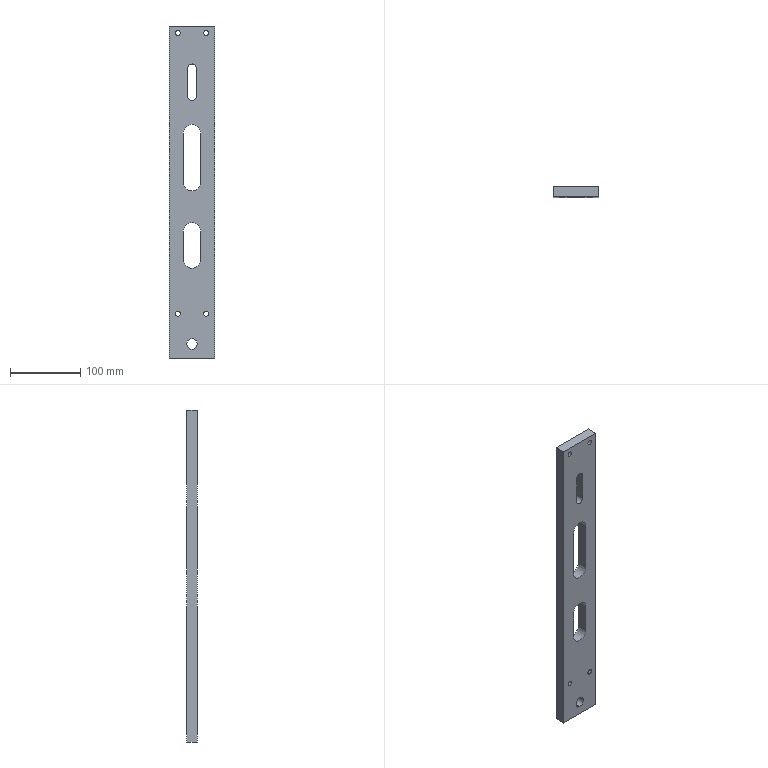Component | SolidWorks | TractionUpperPlate-2 | 1 solid | 31 faces | box 65 x 15 x 473 mm | volume 391343 mm3 | cylinder 19 | plane 12 | commonest cylinder face diameters 7 x8 25 x6 12 x3 15 x2
build123d program:
from build123d import *

# Parameters (mm, degrees)
SKETCH1_W      = 473
SKETCH1_H      = 65
SKETCH1_R      = 3.5
SKETCH1_R_2    = 7.5
EXTRUDE1_DEPTH = 15


with BuildPart() as part:
    # Sketch1 → Extrude1 (new body)
    with BuildSketch(Plane.XY):
        Rectangle(SKETCH1_W, SKETCH1_H)
        with Locations((-226.5, 20)):
            Circle(SKETCH1_R, mode=Mode.SUBTRACT)
        with Locations((-226.5, -20)):
            Circle(SKETCH1_R, mode=Mode.SUBTRACT)
        with Locations((173.5, 20)):
            Circle(SKETCH1_R, mode=Mode.SUBTRACT)
        with Locations((173.5, -20)):
            Circle(SKETCH1_R, mode=Mode.SUBTRACT)
        with Locations((216.5, 0)):
            Circle(SKETCH1_R_2, mode=Mode.SUBTRACT)
        with BuildLine():
            Line((-176.5, 6), (-136.5, 6))
            ThreePointArc((-136.5, 6), (-130.5, 0), (-136.5, -6))
            Line((-136.5, -6), (-176.5, -6))
            ThreePointArc((-176.5, -6), (-182.5, 0), (-176.5, 6))
        make_face(mode=Mode.SUBTRACT)
        with BuildLine():
            Line((-84, 12.5), (-14, 12.5))
            ThreePointArc((-14, 12.5), (-1.5, 0), (-14, -12.5))
            Line((-14, -12.5), (-84, -12.5))
            ThreePointArc((-84, -12.5), (-96.5, 0), (-84, 12.5))
        make_face(mode=Mode.SUBTRACT)
        with BuildLine():
            Line((56, 12.5), (96, 12.5))
            ThreePointArc((96, 12.5), (108.5, 0), (96, -12.5))
            Line((96, -12.5), (56, -12.5))
            ThreePointArc((56, -12.5), (43.5, 0), (56, 12.5))
        make_face(mode=Mode.SUBTRACT)
    extrude(amount=EXTRUDE1_DEPTH)


solid = part.part

# Placed as in the assembly
solid = solid.moved(Location((250.216, 526.983, 40), (90, 0, -90)))
STEP:
#1=CARTESIAN_POINT('',(9.851,20.157,-6.654));
#2=VERTEX_POINT('',#1);
#3=CARTESIAN_POINT('',(9.851,20.157,-7.244));
#4=VERTEX_POINT('',#3);
#5=CARTESIAN_POINT('',(9.851,20.157,-6.949));
#6=DIRECTION('',(0.,-1.,0.));
#7=DIRECTION('',(0.,0.,-1.));
#8=AXIS2_PLACEMENT_3D('',#5,#6,#7);
#9=CIRCLE('',#8,0.2953);
#10=EDGE_CURVE('',#2,#4,#9,.T.);
#11=ORIENTED_EDGE('',*,*,#10,.T.);
#12=CARTESIAN_POINT('',(9.851,20.747,-7.244));
#13=VERTEX_POINT('',#12);
#14=CARTESIAN_POINT('',(9.851,20.157,-7.244));
#15=DIRECTION('',(0.,1.,0.));
#16=VECTOR('',#15,39.37);
#17=LINE('',#14,#16);
#18=EDGE_CURVE('',#4,#13,#17,.T.);
#19=ORIENTED_EDGE('',*,*,#18,.T.);
#20=CARTESIAN_POINT('',(9.851,20.747,-6.654));
#21=VERTEX_POINT('',#20);
#22=CARTESIAN_POINT('',(9.851,20.747,-6.949));
#23=DIRECTION('',(0.,-1.,0.));
#24=DIRECTION('',(0.,0.,-1.));
#25=AXIS2_PLACEMENT_3D('',#22,#23,#24);
#26=CIRCLE('',#25,0.2953);
#27=EDGE_CURVE('',#21,#13,#26,.T.);
#28=ORIENTED_EDGE('',*,*,#27,.F.);
#29=CARTESIAN_POINT('',(9.851,20.157,-6.654));
#30=DIRECTION('',(0.,1.,0.));
#31=VECTOR('',#30,39.37);
#32=LINE('',#29,#31);
#33=EDGE_CURVE('',#2,#21,#32,.T.);
#34=ORIENTED_EDGE('',*,*,#33,.F.);
#35=EDGE_LOOP('',(#11,#19,#28,#34));
#36=FACE_OUTER_BOUND('',#35,.T.);
#37=CARTESIAN_POINT('',(9.851,20.157,-6.949));
#38=DIRECTION('',(0.,1.,0.));
#39=DIRECTION('',(0.,0.,1.));
#40=AXIS2_PLACEMENT_3D('',#37,#38,#39);
#41=CYLINDRICAL_SURFACE('',#40,0.2953);
#42=ADVANCED_FACE('',(#36),#41,.F.);
#43=CARTESIAN_POINT('',(9.064,20.157,-5.118));
#44=VERTEX_POINT('',#43);
#45=CARTESIAN_POINT('',(9.064,20.157,-5.394));
#46=VERTEX_POINT('',#45);
#47=CARTESIAN_POINT('',(9.064,20.157,-5.256));
#48=DIRECTION('',(0.,-1.,0.));
#49=DIRECTION('',(0.,0.,-1.));
#50=AXIS2_PLACEMENT_3D('',#47,#48,#49);
#51=CIRCLE('',#50,0.1378);
#52=EDGE_CURVE('',#44,#46,#51,.T.);
#53=ORIENTED_EDGE('',*,*,#52,.T.);
#54=CARTESIAN_POINT('',(9.064,20.747,-5.394));
#55=VERTEX_POINT('',#54);
#56=CARTESIAN_POINT('',(9.064,20.157,-5.394));
#57=DIRECTION('',(0.,1.,0.));
#58=VECTOR('',#57,39.37);
#59=LINE('',#56,#58);
#60=EDGE_CURVE('',#46,#55,#59,.T.);
#61=ORIENTED_EDGE('',*,*,#60,.T.);
#62=CARTESIAN_POINT('',(9.064,20.747,-5.118));
#63=VERTEX_POINT('',#62);
#64=CARTESIAN_POINT('',(9.064,20.747,-5.256));
#65=DIRECTION('',(0.,-1.,0.));
#66=DIRECTION('',(0.,0.,-1.));
#67=AXIS2_PLACEMENT_3D('',#64,#65,#66);
#68=CIRCLE('',#67,0.1378);
#69=EDGE_CURVE('',#63,#55,#68,.T.);
#70=ORIENTED_EDGE('',*,*,#69,.F.);
#71=CARTESIAN_POINT('',(9.064,20.157,-5.118));
#72=DIRECTION('',(0.,1.,0.));
#73=VECTOR('',#72,39.37);
#74=LINE('',#71,#73);
#75=EDGE_CURVE('',#44,#63,#74,.T.);
#76=ORIENTED_EDGE('',*,*,#75,.F.);
#77=EDGE_LOOP('',(#53,#61,#70,#76));
#78=FACE_OUTER_BOUND('',#77,.T.);
#79=CARTESIAN_POINT('',(9.064,20.157,-5.256));
#80=DIRECTION('',(0.,1.,0.));
#81=DIRECTION('',(0.,0.,1.));
#82=AXIS2_PLACEMENT_3D('',#79,#80,#81);
#83=CYLINDRICAL_SURFACE('',#82,0.1378);
#84=ADVANCED_FACE('',(#78),#83,.F.);
#85=CARTESIAN_POINT('',(10.638,20.157,-5.118));
#86=VERTEX_POINT('',#85);
#87=CARTESIAN_POINT('',(10.638,20.157,-5.394));
#88=VERTEX_POINT('',#87);
#89=CARTESIAN_POINT('',(10.638,20.157,-5.256));
#90=DIRECTION('',(0.,-1.,0.));
#91=DIRECTION('',(0.,0.,-1.));
#92=AXIS2_PLACEMENT_3D('',#89,#90,#91);
#93=CIRCLE('',#92,0.1378);
#94=EDGE_CURVE('',#86,#88,#93,.T.);
#95=ORIENTED_EDGE('',*,*,#94,.T.);
#96=CARTESIAN_POINT('',(10.638,20.747,-5.394));
#97=VERTEX_POINT('',#96);
#98=CARTESIAN_POINT('',(10.638,20.157,-5.394));
#99=DIRECTION('',(0.,1.,0.));
#100=VECTOR('',#99,39.37);
#101=LINE('',#98,#100);
#102=EDGE_CURVE('',#88,#97,#101,.T.);
#103=ORIENTED_EDGE('',*,*,#102,.T.);
#104=CARTESIAN_POINT('',(10.638,20.747,-5.118));
#105=VERTEX_POINT('',#104);
#106=CARTESIAN_POINT('',(10.638,20.747,-5.256));
#107=DIRECTION('',(0.,-1.,0.));
#108=DIRECTION('',(0.,0.,-1.));
#109=AXIS2_PLACEMENT_3D('',#106,#107,#108);
#110=CIRCLE('',#109,0.1378);
#111=EDGE_CURVE('',#105,#97,#110,.T.);
#112=ORIENTED_EDGE('',*,*,#111,.F.);
#113=CARTESIAN_POINT('',(10.638,20.157,-5.118));
#114=DIRECTION('',(0.,1.,0.));
#115=VECTOR('',#114,39.37);
#116=LINE('',#113,#115);
#117=EDGE_CURVE('',#86,#105,#116,.T.);
#118=ORIENTED_EDGE('',*,*,#117,.F.);
#119=EDGE_LOOP('',(#95,#103,#112,#118));
#120=FACE_OUTER_BOUND('',#119,.T.);
#121=CARTESIAN_POINT('',(10.638,20.157,-5.256));
#122=DIRECTION('',(0.,1.,0.));
#123=DIRECTION('',(0.,0.,1.));
#124=AXIS2_PLACEMENT_3D('',#121,#122,#123);
#125=CYLINDRICAL_SURFACE('',#124,0.1378);
#126=ADVANCED_FACE('',(#120),#125,.F.);
#127=CARTESIAN_POINT('',(10.343,20.157,-0.6299));
#128=VERTEX_POINT('',#127);
#129=CARTESIAN_POINT('',(9.851,20.157,-0.1378));
#130=VERTEX_POINT('',#129);
#131=CARTESIAN_POINT('',(9.851,20.157,-0.6299));
#132=DIRECTION('',(0.,-1.,0.));
#133=DIRECTION('',(0.,0.,-1.));
#134=AXIS2_PLACEMENT_3D('',#131,#132,#133);
#135=CIRCLE('',#134,0.4921);
#136=EDGE_CURVE('',#128,#130,#135,.T.);
#137=ORIENTED_EDGE('',*,*,#136,.T.);
#138=CARTESIAN_POINT('',(9.851,20.747,-0.1378));
#139=VERTEX_POINT('',#138);
#140=CARTESIAN_POINT('',(9.851,20.157,-0.1378));
#141=DIRECTION('',(0.,1.,0.));
#142=VECTOR('',#141,39.37);
#143=LINE('',#140,#142);
#144=EDGE_CURVE('',#130,#139,#143,.T.);
#145=ORIENTED_EDGE('',*,*,#144,.T.);
#146=CARTESIAN_POINT('',(10.343,20.747,-0.6299));
#147=VERTEX_POINT('',#146);
#148=CARTESIAN_POINT('',(9.851,20.747,-0.6299));
#149=DIRECTION('',(0.,-1.,0.));
#150=DIRECTION('',(0.,0.,-1.));
#151=AXIS2_PLACEMENT_3D('',#148,#149,#150);
#152=CIRCLE('',#151,0.4921);
#153=EDGE_CURVE('',#147,#139,#152,.T.);
#154=ORIENTED_EDGE('',*,*,#153,.F.);
#155=CARTESIAN_POINT('',(10.343,20.157,-0.6299));
#156=DIRECTION('',(0.,1.,0.));
#157=VECTOR('',#156,39.37);
#158=LINE('',#155,#157);
#159=EDGE_CURVE('',#128,#147,#158,.T.);
#160=ORIENTED_EDGE('',*,*,#159,.F.);
#161=EDGE_LOOP('',(#137,#145,#154,#160));
#162=FACE_OUTER_BOUND('',#161,.T.);
#163=CARTESIAN_POINT('',(9.851,20.157,-0.6299));
#164=DIRECTION('',(0.,1.,0.));
#165=DIRECTION('',(0.,0.,1.));
#166=AXIS2_PLACEMENT_3D('',#163,#164,#165);
#167=CYLINDRICAL_SURFACE('',#166,0.4921);
#168=ADVANCED_FACE('',(#162),#167,.F.);
#169=CARTESIAN_POINT('',(10.343,20.157,4.882));
#170=VERTEX_POINT('',#169);
#171=CARTESIAN_POINT('',(9.851,20.157,5.374));
#172=VERTEX_POINT('',#171);
#173=CARTESIAN_POINT('',(9.851,20.157,4.882));
#174=DIRECTION('',(0.,-1.,0.));
#175=DIRECTION('',(0.,0.,-1.));
#176=AXIS2_PLACEMENT_3D('',#173,#174,#175);
#177=CIRCLE('',#176,0.4921);
#178=EDGE_CURVE('',#170,#172,#177,.T.);
#179=ORIENTED_EDGE('',*,*,#178,.T.);
#180=CARTESIAN_POINT('',(9.851,20.747,5.374));
#181=VERTEX_POINT('',#180);
#182=CARTESIAN_POINT('',(9.851,20.157,5.374));
#183=DIRECTION('',(0.,1.,0.));
#184=VECTOR('',#183,39.37);
#185=LINE('',#182,#184);
#186=EDGE_CURVE('',#172,#181,#185,.T.);
#187=ORIENTED_EDGE('',*,*,#186,.T.);
#188=CARTESIAN_POINT('',(10.343,20.747,4.882));
#189=VERTEX_POINT('',#188);
#190=CARTESIAN_POINT('',(9.851,20.747,4.882));
#191=DIRECTION('',(0.,-1.,0.));
#192=DIRECTION('',(0.,0.,-1.));
#193=AXIS2_PLACEMENT_3D('',#190,#191,#192);
#194=CIRCLE('',#193,0.4921);
#195=EDGE_CURVE('',#189,#181,#194,.T.);
#196=ORIENTED_EDGE('',*,*,#195,.F.);
#197=CARTESIAN_POINT('',(10.343,20.157,4.882));
#198=DIRECTION('',(0.,1.,0.));
#199=VECTOR('',#198,39.37);
#200=LINE('',#197,#199);
#201=EDGE_CURVE('',#170,#189,#200,.T.);
#202=ORIENTED_EDGE('',*,*,#201,.F.);
#203=EDGE_LOOP('',(#179,#187,#196,#202));
#204=FACE_OUTER_BOUND('',#203,.T.);
#205=CARTESIAN_POINT('',(9.851,20.157,4.882));
#206=DIRECTION('',(0.,1.,0.));
#207=DIRECTION('',(0.,0.,1.));
#208=AXIS2_PLACEMENT_3D('',#205,#206,#207);
#209=CYLINDRICAL_SURFACE('',#208,0.4921);
#210=ADVANCED_FACE('',(#204),#209,.F.);
#211=CARTESIAN_POINT('',(9.064,20.157,10.63));
#212=VERTEX_POINT('',#211);
#213=CARTESIAN_POINT('',(9.064,20.157,10.354));
#214=VERTEX_POINT('',#213);
#215=CARTESIAN_POINT('',(9.064,20.157,10.492));
#216=DIRECTION('',(0.,-1.,0.));
#217=DIRECTION('',(0.,0.,-1.));
#218=AXIS2_PLACEMENT_3D('',#215,#216,#217);
#219=CIRCLE('',#218,0.1378);
#220=EDGE_CURVE('',#212,#214,#219,.T.);
#221=ORIENTED_EDGE('',*,*,#220,.T.);
#222=CARTESIAN_POINT('',(9.064,20.747,10.354));
#223=VERTEX_POINT('',#222);
#224=CARTESIAN_POINT('',(9.064,20.157,10.354));
#225=DIRECTION('',(0.,1.,0.));
#226=VECTOR('',#225,39.37);
#227=LINE('',#224,#226);
#228=EDGE_CURVE('',#214,#223,#227,.T.);
#229=ORIENTED_EDGE('',*,*,#228,.T.);
#230=CARTESIAN_POINT('',(9.064,20.747,10.63));
#231=VERTEX_POINT('',#230);
#232=CARTESIAN_POINT('',(9.064,20.747,10.492));
#233=DIRECTION('',(0.,-1.,0.));
#234=DIRECTION('',(0.,0.,-1.));
#235=AXIS2_PLACEMENT_3D('',#232,#233,#234);
#236=CIRCLE('',#235,0.1378);
#237=EDGE_CURVE('',#231,#223,#236,.T.);
#238=ORIENTED_EDGE('',*,*,#237,.F.);
#239=CARTESIAN_POINT('',(9.064,20.157,10.63));
#240=DIRECTION('',(0.,1.,0.));
#241=VECTOR('',#240,39.37);
#242=LINE('',#239,#241);
#243=EDGE_CURVE('',#212,#231,#242,.T.);
#244=ORIENTED_EDGE('',*,*,#243,.F.);
#245=EDGE_LOOP('',(#221,#229,#238,#244));
#246=FACE_OUTER_BOUND('',#245,.T.);
#247=CARTESIAN_POINT('',(9.064,20.157,10.492));
#248=DIRECTION('',(0.,1.,0.));
#249=DIRECTION('',(0.,0.,1.));
#250=AXIS2_PLACEMENT_3D('',#247,#248,#249);
#251=CYLINDRICAL_SURFACE('',#250,0.1378);
#252=ADVANCED_FACE('',(#246),#251,.F.);
#253=CARTESIAN_POINT('',(10.638,20.157,10.63));
#254=VERTEX_POINT('',#253);
#255=CARTESIAN_POINT('',(10.638,20.157,10.354));
#256=VERTEX_POINT('',#255);
#257=CARTESIAN_POINT('',(10.638,20.157,10.492));
#258=DIRECTION('',(0.,-1.,0.));
#259=DIRECTION('',(0.,0.,-1.));
#260=AXIS2_PLACEMENT_3D('',#257,#258,#259);
#261=CIRCLE('',#260,0.1378);
#262=EDGE_CURVE('',#254,#256,#261,.T.);
#263=ORIENTED_EDGE('',*,*,#262,.T.);
#264=CARTESIAN_POINT('',(10.638,20.747,10.354));
#265=VERTEX_POINT('',#264);
#266=CARTESIAN_POINT('',(10.638,20.157,10.354));
#267=DIRECTION('',(0.,1.,0.));
#268=VECTOR('',#267,39.37);
#269=LINE('',#266,#268);
#270=EDGE_CURVE('',#256,#265,#269,.T.);
#271=ORIENTED_EDGE('',*,*,#270,.T.);
#272=CARTESIAN_POINT('',(10.638,20.747,10.63));
#273=VERTEX_POINT('',#272);
#274=CARTESIAN_POINT('',(10.638,20.747,10.492));
#275=DIRECTION('',(0.,-1.,0.));
#276=DIRECTION('',(0.,0.,-1.));
#277=AXIS2_PLACEMENT_3D('',#274,#275,#276);
#278=CIRCLE('',#277,0.1378);
#279=EDGE_CURVE('',#273,#265,#278,.T.);
#280=ORIENTED_EDGE('',*,*,#279,.F.);
#281=CARTESIAN_POINT('',(10.638,20.157,10.63));
#282=DIRECTION('',(0.,1.,0.));
#283=VECTOR('',#282,39.37);
#284=LINE('',#281,#283);
#285=EDGE_CURVE('',#254,#273,#284,.T.);
#286=ORIENTED_EDGE('',*,*,#285,.F.);
#287=EDGE_LOOP('',(#263,#271,#280,#286));
#288=FACE_OUTER_BOUND('',#287,.T.);
#289=CARTESIAN_POINT('',(10.638,20.157,10.492));
#290=DIRECTION('',(0.,1.,0.));
#291=DIRECTION('',(0.,0.,1.));
#292=AXIS2_PLACEMENT_3D('',#289,#290,#291);
#293=CYLINDRICAL_SURFACE('',#292,0.1378);
#294=ADVANCED_FACE('',(#288),#293,.F.);
#295=CARTESIAN_POINT('',(10.087,20.157,8.524));
#296=VERTEX_POINT('',#295);
#297=CARTESIAN_POINT('',(9.851,20.157,8.76));
#298=VERTEX_POINT('',#297);
#299=CARTESIAN_POINT('',(9.851,20.157,8.524));
#300=DIRECTION('',(0.,-1.,0.));
#301=DIRECTION('',(0.,0.,-1.));
#302=AXIS2_PLACEMENT_3D('',#299,#300,#301);
#303=CIRCLE('',#302,0.2362);
#304=EDGE_CURVE('',#296,#298,#303,.T.);
#305=ORIENTED_EDGE('',*,*,#304,.T.);
#306=CARTESIAN_POINT('',(9.851,20.747,8.76));
#307=VERTEX_POINT('',#306);
#308=CARTESIAN_POINT('',(9.851,20.157,8.76));
#309=DIRECTION('',(0.,1.,0.));
#310=VECTOR('',#309,39.37);
#311=LINE('',#308,#310);
#312=EDGE_CURVE('',#298,#307,#311,.T.);
#313=ORIENTED_EDGE('',*,*,#312,.T.);
#314=CARTESIAN_POINT('',(10.087,20.747,8.524));
#315=VERTEX_POINT('',#314);
#316=CARTESIAN_POINT('',(9.851,20.747,8.524));
#317=DIRECTION('',(0.,-1.,0.));
#318=DIRECTION('',(0.,0.,-1.));
#319=AXIS2_PLACEMENT_3D('',#316,#317,#318);
#320=CIRCLE('',#319,0.2362);
#321=EDGE_CURVE('',#315,#307,#320,.T.);
#322=ORIENTED_EDGE('',*,*,#321,.F.);
#323=CARTESIAN_POINT('',(10.087,20.157,8.524));
#324=DIRECTION('',(0.,1.,0.));
#325=VECTOR('',#324,39.37);
#326=LINE('',#323,#325);
#327=EDGE_CURVE('',#296,#315,#326,.T.);
#328=ORIENTED_EDGE('',*,*,#327,.F.);
#329=EDGE_LOOP('',(#305,#313,#322,#328));
#330=FACE_OUTER_BOUND('',#329,.T.);
#331=CARTESIAN_POINT('',(9.851,20.157,8.524));
#332=DIRECTION('',(0.,1.,0.));
#333=DIRECTION('',(0.,0.,1.));
#334=AXIS2_PLACEMENT_3D('',#331,#332,#333);
#335=CYLINDRICAL_SURFACE('',#334,0.2362);
#336=ADVANCED_FACE('',(#330),#335,.F.);
#337=ORIENTED_EDGE('',*,*,#52,.F.);
#338=CARTESIAN_POINT('',(9.064,20.157,-5.256));
#339=DIRECTION('',(0.,-1.,0.));
#340=DIRECTION('',(0.,0.,-1.));
#341=AXIS2_PLACEMENT_3D('',#338,#339,#340);
#342=CIRCLE('',#341,0.1378);
#343=EDGE_CURVE('',#46,#44,#342,.T.);
#344=ORIENTED_EDGE('',*,*,#343,.F.);
#345=EDGE_LOOP('',(#337,#344));
#346=FACE_BOUND('',#345,.T.);
#347=CARTESIAN_POINT('',(9.359,20.157,-0.6299));
#348=VERTEX_POINT('',#347);
#349=CARTESIAN_POINT('',(9.359,20.157,-2.205));
#350=VERTEX_POINT('',#349);
#351=CARTESIAN_POINT('',(9.359,20.157,-0.6299));
#352=DIRECTION('',(0.,0.,-1.));
#353=VECTOR('',#352,39.37);
#354=LINE('',#351,#353);
#355=EDGE_CURVE('',#348,#350,#354,.T.);
#356=ORIENTED_EDGE('',*,*,#355,.F.);
#357=CARTESIAN_POINT('',(9.851,20.157,-0.6299));
#358=DIRECTION('',(0.,-1.,0.));
#359=DIRECTION('',(0.,0.,-1.));
#360=AXIS2_PLACEMENT_3D('',#357,#358,#359);
#361=CIRCLE('',#360,0.4921);
#362=EDGE_CURVE('',#130,#348,#361,.T.);
#363=ORIENTED_EDGE('',*,*,#362,.F.);
#364=ORIENTED_EDGE('',*,*,#136,.F.);
#365=CARTESIAN_POINT('',(10.343,20.157,-2.205));
#366=VERTEX_POINT('',#365);
#367=CARTESIAN_POINT('',(10.343,20.157,-0.6299));
#368=DIRECTION('',(-0.,0.,1.));
#369=VECTOR('',#368,39.37);
#370=LINE('',#367,#369);
#371=EDGE_CURVE('',#366,#128,#370,.T.);
#372=ORIENTED_EDGE('',*,*,#371,.F.);
#373=CARTESIAN_POINT('',(9.851,20.157,-2.205));
#374=DIRECTION('',(0.,-1.,0.));
#375=DIRECTION('',(0.,0.,-1.));
#376=AXIS2_PLACEMENT_3D('',#373,#374,#375);
#377=CIRCLE('',#376,0.4921);
#378=EDGE_CURVE('',#350,#366,#377,.T.);
#379=ORIENTED_EDGE('',*,*,#378,.F.);
#380=EDGE_LOOP('',(#356,#363,#364,#372,#379));
#381=FACE_BOUND('',#380,.T.);
#382=CARTESIAN_POINT('',(9.359,20.157,4.882));
#383=VERTEX_POINT('',#382);
#384=CARTESIAN_POINT('',(9.359,20.157,2.126));
#385=VERTEX_POINT('',#384);
#386=CARTESIAN_POINT('',(9.359,20.157,4.882));
#387=DIRECTION('',(0.,0.,-1.));
#388=VECTOR('',#387,39.37);
#389=LINE('',#386,#388);
#390=EDGE_CURVE('',#383,#385,#389,.T.);
#391=ORIENTED_EDGE('',*,*,#390,.F.);
#392=CARTESIAN_POINT('',(9.851,20.157,4.882));
#393=DIRECTION('',(0.,-1.,0.));
#394=DIRECTION('',(0.,0.,-1.));
#395=AXIS2_PLACEMENT_3D('',#392,#393,#394);
#396=CIRCLE('',#395,0.4921);
#397=EDGE_CURVE('',#172,#383,#396,.T.);
#398=ORIENTED_EDGE('',*,*,#397,.F.);
#399=ORIENTED_EDGE('',*,*,#178,.F.);
#400=CARTESIAN_POINT('',(10.343,20.157,2.126));
#401=VERTEX_POINT('',#400);
#402=CARTESIAN_POINT('',(10.343,20.157,4.882));
#403=DIRECTION('',(-0.,0.,1.));
#404=VECTOR('',#403,39.37);
#405=LINE('',#402,#404);
#406=EDGE_CURVE('',#401,#170,#405,.T.);
#407=ORIENTED_EDGE('',*,*,#406,.F.);
#408=CARTESIAN_POINT('',(9.851,20.157,2.126));
#409=DIRECTION('',(0.,-1.,0.));
#410=DIRECTION('',(0.,0.,-1.));
#411=AXIS2_PLACEMENT_3D('',#408,#409,#410);
#412=CIRCLE('',#411,0.4921);
#413=EDGE_CURVE('',#385,#401,#412,.T.);
#414=ORIENTED_EDGE('',*,*,#413,.F.);
#415=EDGE_LOOP('',(#391,#398,#399,#407,#414));
#416=FACE_BOUND('',#415,.T.);
#417=ORIENTED_EDGE('',*,*,#220,.F.);
#418=CARTESIAN_POINT('',(9.064,20.157,10.492));
#419=DIRECTION('',(0.,-1.,0.));
#420=DIRECTION('',(0.,0.,-1.));
#421=AXIS2_PLACEMENT_3D('',#418,#419,#420);
#422=CIRCLE('',#421,0.1378);
#423=EDGE_CURVE('',#214,#212,#422,.T.);
#424=ORIENTED_EDGE('',*,*,#423,.F.);
#425=EDGE_LOOP('',(#417,#424));
#426=FACE_BOUND('',#425,.T.);
#427=CARTESIAN_POINT('',(9.615,20.157,8.524));
#428=VERTEX_POINT('',#427);
#429=CARTESIAN_POINT('',(9.615,20.157,6.949));
#430=VERTEX_POINT('',#429);
#431=CARTESIAN_POINT('',(9.615,20.157,8.524));
#432=DIRECTION('',(0.,0.,-1.));
#433=VECTOR('',#432,39.37);
#434=LINE('',#431,#433);
#435=EDGE_CURVE('',#428,#430,#434,.T.);
#436=ORIENTED_EDGE('',*,*,#435,.F.);
#437=CARTESIAN_POINT('',(9.851,20.157,8.524));
#438=DIRECTION('',(0.,-1.,0.));
#439=DIRECTION('',(0.,0.,-1.));
#440=AXIS2_PLACEMENT_3D('',#437,#438,#439);
#441=CIRCLE('',#440,0.2362);
#442=EDGE_CURVE('',#298,#428,#441,.T.);
#443=ORIENTED_EDGE('',*,*,#442,.F.);
#444=ORIENTED_EDGE('',*,*,#304,.F.);
#445=CARTESIAN_POINT('',(10.087,20.157,6.949));
#446=VERTEX_POINT('',#445);
#447=CARTESIAN_POINT('',(10.087,20.157,8.524));
#448=DIRECTION('',(-0.,0.,1.));
#449=VECTOR('',#448,39.37);
#450=LINE('',#447,#449);
#451=EDGE_CURVE('',#446,#296,#450,.T.);
#452=ORIENTED_EDGE('',*,*,#451,.F.);
#453=CARTESIAN_POINT('',(9.851,20.157,6.949));
#454=DIRECTION('',(0.,-1.,0.));
#455=DIRECTION('',(0.,0.,-1.));
#456=AXIS2_PLACEMENT_3D('',#453,#454,#455);
#457=CIRCLE('',#456,0.2362);
#458=EDGE_CURVE('',#430,#446,#457,.T.);
#459=ORIENTED_EDGE('',*,*,#458,.F.);
#460=EDGE_LOOP('',(#436,#443,#444,#452,#459));
#461=FACE_BOUND('',#460,.T.);
#462=CARTESIAN_POINT('',(11.131,20.157,10.886));
#463=VERTEX_POINT('',#462);
#464=CARTESIAN_POINT('',(8.572,20.157,10.886));
#465=VERTEX_POINT('',#464);
#466=CARTESIAN_POINT('',(11.131,20.157,10.886));
#467=DIRECTION('',(-1.,0.,-0.));
#468=VECTOR('',#467,39.37);
#469=LINE('',#466,#468);
#470=EDGE_CURVE('',#463,#465,#469,.T.);
#471=ORIENTED_EDGE('',*,*,#470,.T.);
#472=CARTESIAN_POINT('',(8.572,20.157,-7.736));
#473=VERTEX_POINT('',#472);
#474=CARTESIAN_POINT('',(8.572,20.157,10.886));
#475=DIRECTION('',(0.,0.,-1.));
#476=VECTOR('',#475,39.37);
#477=LINE('',#474,#476);
#478=EDGE_CURVE('',#465,#473,#477,.T.);
#479=ORIENTED_EDGE('',*,*,#478,.T.);
#480=CARTESIAN_POINT('',(11.131,20.157,-7.736));
#481=VERTEX_POINT('',#480);
#482=CARTESIAN_POINT('',(11.131,20.157,-7.736));
#483=DIRECTION('',(1.,0.,0.));
#484=VECTOR('',#483,39.37);
#485=LINE('',#482,#484);
#486=EDGE_CURVE('',#473,#481,#485,.T.);
#487=ORIENTED_EDGE('',*,*,#486,.T.);
#488=CARTESIAN_POINT('',(11.131,20.157,10.886));
#489=DIRECTION('',(-0.,0.,1.));
#490=VECTOR('',#489,39.37);
#491=LINE('',#488,#490);
#492=EDGE_CURVE('',#481,#463,#491,.T.);
#493=ORIENTED_EDGE('',*,*,#492,.T.);
#494=EDGE_LOOP('',(#471,#479,#487,#493));
#495=FACE_OUTER_BOUND('',#494,.T.);
#496=ORIENTED_EDGE('',*,*,#262,.F.);
#497=CARTESIAN_POINT('',(10.638,20.157,10.492));
#498=DIRECTION('',(0.,-1.,0.));
#499=DIRECTION('',(0.,0.,-1.));
#500=AXIS2_PLACEMENT_3D('',#497,#498,#499);
#501=CIRCLE('',#500,0.1378);
#502=EDGE_CURVE('',#256,#254,#501,.T.);
#503=ORIENTED_EDGE('',*,*,#502,.F.);
#504=EDGE_LOOP('',(#496,#503));
#505=FACE_BOUND('',#504,.T.);
#506=ORIENTED_EDGE('',*,*,#94,.F.);
#507=CARTESIAN_POINT('',(10.638,20.157,-5.256));
#508=DIRECTION('',(0.,-1.,0.));
#509=DIRECTION('',(0.,0.,-1.));
#510=AXIS2_PLACEMENT_3D('',#507,#508,#509);
#511=CIRCLE('',#510,0.1378);
#512=EDGE_CURVE('',#88,#86,#511,.T.);
#513=ORIENTED_EDGE('',*,*,#512,.F.);
#514=EDGE_LOOP('',(#506,#513));
#515=FACE_BOUND('',#514,.T.);
#516=ORIENTED_EDGE('',*,*,#10,.F.);
#517=CARTESIAN_POINT('',(9.851,20.157,-6.949));
#518=DIRECTION('',(0.,-1.,0.));
#519=DIRECTION('',(0.,0.,-1.));
#520=AXIS2_PLACEMENT_3D('',#517,#518,#519);
#521=CIRCLE('',#520,0.2953);
#522=EDGE_CURVE('',#4,#2,#521,.T.);
#523=ORIENTED_EDGE('',*,*,#522,.F.);
#524=EDGE_LOOP('',(#516,#523));
#525=FACE_BOUND('',#524,.T.);
#526=CARTESIAN_POINT('',(8.572,20.157,10.886));
#527=DIRECTION('',(0.,-1.,0.));
#528=DIRECTION('',(0.,0.,-1.));
#529=AXIS2_PLACEMENT_3D('',#526,#527,#528);
#530=PLANE('',#529);
#531=ADVANCED_FACE('',(#346,#381,#416,#426,#461,#495,#505,#515,#525),#530,.T.);
#532=ORIENTED_EDGE('',*,*,#195,.T.);
#533=CARTESIAN_POINT('',(9.359,20.747,4.882));
#534=VERTEX_POINT('',#533);
#535=CARTESIAN_POINT('',(9.851,20.747,4.882));
#536=DIRECTION('',(0.,-1.,0.));
#537=DIRECTION('',(0.,0.,-1.));
#538=AXIS2_PLACEMENT_3D('',#535,#536,#537);
#539=CIRCLE('',#538,0.4921);
#540=EDGE_CURVE('',#181,#534,#539,.T.);
#541=ORIENTED_EDGE('',*,*,#540,.T.);
#542=CARTESIAN_POINT('',(9.359,20.747,2.126));
#543=VERTEX_POINT('',#542);
#544=CARTESIAN_POINT('',(9.359,20.747,4.882));
#545=DIRECTION('',(0.,0.,-1.));
#546=VECTOR('',#545,39.37);
#547=LINE('',#544,#546);
#548=EDGE_CURVE('',#534,#543,#547,.T.);
#549=ORIENTED_EDGE('',*,*,#548,.T.);
#550=CARTESIAN_POINT('',(10.343,20.747,2.126));
#551=VERTEX_POINT('',#550);
#552=CARTESIAN_POINT('',(9.851,20.747,2.126));
#553=DIRECTION('',(0.,-1.,0.));
#554=DIRECTION('',(0.,0.,-1.));
#555=AXIS2_PLACEMENT_3D('',#552,#553,#554);
#556=CIRCLE('',#555,0.4921);
#557=EDGE_CURVE('',#543,#551,#556,.T.);
#558=ORIENTED_EDGE('',*,*,#557,.T.);
#559=CARTESIAN_POINT('',(10.343,20.747,4.882));
#560=DIRECTION('',(-0.,0.,1.));
#561=VECTOR('',#560,39.37);
#562=LINE('',#559,#561);
#563=EDGE_CURVE('',#551,#189,#562,.T.);
#564=ORIENTED_EDGE('',*,*,#563,.T.);
#565=EDGE_LOOP('',(#532,#541,#549,#558,#564));
#566=FACE_BOUND('',#565,.T.);
#567=CARTESIAN_POINT('',(11.131,20.747,10.886));
#568=VERTEX_POINT('',#567);
#569=CARTESIAN_POINT('',(8.572,20.747,10.886));
#570=VERTEX_POINT('',#569);
#571=CARTESIAN_POINT('',(11.131,20.747,10.886));
#572=DIRECTION('',(-1.,0.,-0.));
#573=VECTOR('',#572,39.37);
#574=LINE('',#571,#573);
#575=EDGE_CURVE('',#568,#570,#574,.T.);
#576=ORIENTED_EDGE('',*,*,#575,.F.);
#577=CARTESIAN_POINT('',(11.131,20.747,-7.736));
#578=VERTEX_POINT('',#577);
#579=CARTESIAN_POINT('',(11.131,20.747,10.886));
#580=DIRECTION('',(-0.,0.,1.));
#581=VECTOR('',#580,39.37);
#582=LINE('',#579,#581);
#583=EDGE_CURVE('',#578,#568,#582,.T.);
#584=ORIENTED_EDGE('',*,*,#583,.F.);
#585=CARTESIAN_POINT('',(8.572,20.747,-7.736));
#586=VERTEX_POINT('',#585);
#587=CARTESIAN_POINT('',(11.131,20.747,-7.736));
#588=DIRECTION('',(1.,0.,0.));
#589=VECTOR('',#588,39.37);
#590=LINE('',#587,#589);
#591=EDGE_CURVE('',#586,#578,#590,.T.);
#592=ORIENTED_EDGE('',*,*,#591,.F.);
#593=CARTESIAN_POINT('',(8.572,20.747,10.886));
#594=DIRECTION('',(0.,0.,-1.));
#595=VECTOR('',#594,39.37);
#596=LINE('',#593,#595);
#597=EDGE_CURVE('',#570,#586,#596,.T.);
#598=ORIENTED_EDGE('',*,*,#597,.F.);
#599=EDGE_LOOP('',(#576,#584,#592,#598));
#600=FACE_OUTER_BOUND('',#599,.T.);
#601=ORIENTED_EDGE('',*,*,#321,.T.);
#602=CARTESIAN_POINT('',(9.615,20.747,8.524));
#603=VERTEX_POINT('',#602);
#604=CARTESIAN_POINT('',(9.851,20.747,8.524));
#605=DIRECTION('',(0.,-1.,0.));
#606=DIRECTION('',(0.,0.,-1.));
#607=AXIS2_PLACEMENT_3D('',#604,#605,#606);
#608=CIRCLE('',#607,0.2362);
#609=EDGE_CURVE('',#307,#603,#608,.T.);
#610=ORIENTED_EDGE('',*,*,#609,.T.);
#611=CARTESIAN_POINT('',(9.615,20.747,6.949));
#612=VERTEX_POINT('',#611);
#613=CARTESIAN_POINT('',(9.615,20.747,8.524));
#614=DIRECTION('',(0.,0.,-1.));
#615=VECTOR('',#614,39.37);
#616=LINE('',#613,#615);
#617=EDGE_CURVE('',#603,#612,#616,.T.);
#618=ORIENTED_EDGE('',*,*,#617,.T.);
#619=CARTESIAN_POINT('',(10.087,20.747,6.949));
#620=VERTEX_POINT('',#619);
#621=CARTESIAN_POINT('',(9.851,20.747,6.949));
#622=DIRECTION('',(0.,-1.,0.));
#623=DIRECTION('',(0.,0.,-1.));
#624=AXIS2_PLACEMENT_3D('',#621,#622,#623);
#625=CIRCLE('',#624,0.2362);
#626=EDGE_CURVE('',#612,#620,#625,.T.);
#627=ORIENTED_EDGE('',*,*,#626,.T.);
#628=CARTESIAN_POINT('',(10.087,20.747,8.524));
#629=DIRECTION('',(-0.,0.,1.));
#630=VECTOR('',#629,39.37);
#631=LINE('',#628,#630);
#632=EDGE_CURVE('',#620,#315,#631,.T.);
#633=ORIENTED_EDGE('',*,*,#632,.T.);
#634=EDGE_LOOP('',(#601,#610,#618,#627,#633));
#635=FACE_BOUND('',#634,.T.);
#636=ORIENTED_EDGE('',*,*,#279,.T.);
#637=CARTESIAN_POINT('',(10.638,20.747,10.492));
#638=DIRECTION('',(0.,-1.,0.));
#639=DIRECTION('',(0.,0.,-1.));
#640=AXIS2_PLACEMENT_3D('',#637,#638,#639);
#641=CIRCLE('',#640,0.1378);
#642=EDGE_CURVE('',#265,#273,#641,.T.);
#643=ORIENTED_EDGE('',*,*,#642,.T.);
#644=EDGE_LOOP('',(#636,#643));
#645=FACE_BOUND('',#644,.T.);
#646=ORIENTED_EDGE('',*,*,#237,.T.);
#647=CARTESIAN_POINT('',(9.064,20.747,10.492));
#648=DIRECTION('',(0.,-1.,0.));
#649=DIRECTION('',(0.,0.,-1.));
#650=AXIS2_PLACEMENT_3D('',#647,#648,#649);
#651=CIRCLE('',#650,0.1378);
#652=EDGE_CURVE('',#223,#231,#651,.T.);
#653=ORIENTED_EDGE('',*,*,#652,.T.);
#654=EDGE_LOOP('',(#646,#653));
#655=FACE_BOUND('',#654,.T.);
#656=ORIENTED_EDGE('',*,*,#153,.T.);
#657=CARTESIAN_POINT('',(9.359,20.747,-0.6299));
#658=VERTEX_POINT('',#657);
#659=CARTESIAN_POINT('',(9.851,20.747,-0.6299));
#660=DIRECTION('',(0.,-1.,0.));
#661=DIRECTION('',(0.,0.,-1.));
#662=AXIS2_PLACEMENT_3D('',#659,#660,#661);
#663=CIRCLE('',#662,0.4921);
#664=EDGE_CURVE('',#139,#658,#663,.T.);
#665=ORIENTED_EDGE('',*,*,#664,.T.);
#666=CARTESIAN_POINT('',(9.359,20.747,-2.205));
#667=VERTEX_POINT('',#666);
#668=CARTESIAN_POINT('',(9.359,20.747,-0.6299));
#669=DIRECTION('',(0.,0.,-1.));
#670=VECTOR('',#669,39.37);
#671=LINE('',#668,#670);
#672=EDGE_CURVE('',#658,#667,#671,.T.);
#673=ORIENTED_EDGE('',*,*,#672,.T.);
#674=CARTESIAN_POINT('',(10.343,20.747,-2.205));
#675=VERTEX_POINT('',#674);
#676=CARTESIAN_POINT('',(9.851,20.747,-2.205));
#677=DIRECTION('',(0.,-1.,0.));
#678=DIRECTION('',(0.,0.,-1.));
#679=AXIS2_PLACEMENT_3D('',#676,#677,#678);
#680=CIRCLE('',#679,0.4921);
#681=EDGE_CURVE('',#667,#675,#680,.T.);
#682=ORIENTED_EDGE('',*,*,#681,.T.);
#683=CARTESIAN_POINT('',(10.343,20.747,-0.6299));
#684=DIRECTION('',(-0.,0.,1.));
#685=VECTOR('',#684,39.37);
#686=LINE('',#683,#685);
#687=EDGE_CURVE('',#675,#147,#686,.T.);
#688=ORIENTED_EDGE('',*,*,#687,.T.);
#689=EDGE_LOOP('',(#656,#665,#673,#682,#688));
#690=FACE_BOUND('',#689,.T.);
#691=ORIENTED_EDGE('',*,*,#111,.T.);
#692=CARTESIAN_POINT('',(10.638,20.747,-5.256));
#693=DIRECTION('',(0.,-1.,0.));
#694=DIRECTION('',(0.,0.,-1.));
#695=AXIS2_PLACEMENT_3D('',#692,#693,#694);
#696=CIRCLE('',#695,0.1378);
#697=EDGE_CURVE('',#97,#105,#696,.T.);
#698=ORIENTED_EDGE('',*,*,#697,.T.);
#699=EDGE_LOOP('',(#691,#698));
#700=FACE_BOUND('',#699,.T.);
#701=ORIENTED_EDGE('',*,*,#69,.T.);
#702=CARTESIAN_POINT('',(9.064,20.747,-5.256));
#703=DIRECTION('',(0.,-1.,0.));
#704=DIRECTION('',(0.,0.,-1.));
#705=AXIS2_PLACEMENT_3D('',#702,#703,#704);
#706=CIRCLE('',#705,0.1378);
#707=EDGE_CURVE('',#55,#63,#706,.T.);
#708=ORIENTED_EDGE('',*,*,#707,.T.);
#709=EDGE_LOOP('',(#701,#708));
#710=FACE_BOUND('',#709,.T.);
#711=ORIENTED_EDGE('',*,*,#27,.T.);
#712=CARTESIAN_POINT('',(9.851,20.747,-6.949));
#713=DIRECTION('',(0.,-1.,0.));
#714=DIRECTION('',(0.,0.,-1.));
#715=AXIS2_PLACEMENT_3D('',#712,#713,#714);
#716=CIRCLE('',#715,0.2953);
#717=EDGE_CURVE('',#13,#21,#716,.T.);
#718=ORIENTED_EDGE('',*,*,#717,.T.);
#719=EDGE_LOOP('',(#711,#718));
#720=FACE_BOUND('',#719,.T.);
#721=CARTESIAN_POINT('',(8.572,20.747,10.886));
#722=DIRECTION('',(0.,-1.,0.));
#723=DIRECTION('',(0.,0.,-1.));
#724=AXIS2_PLACEMENT_3D('',#721,#722,#723);
#725=PLANE('',#724);
#726=ADVANCED_FACE('',(#566,#600,#635,#645,#655,#690,#700,#710,#720),#725,.F.);
#727=ORIENTED_EDGE('',*,*,#575,.T.);
#728=CARTESIAN_POINT('',(8.572,20.157,10.886));
#729=DIRECTION('',(0.,1.,0.));
#730=VECTOR('',#729,39.37);
#731=LINE('',#728,#730);
#732=EDGE_CURVE('',#465,#570,#731,.T.);
#733=ORIENTED_EDGE('',*,*,#732,.F.);
#734=ORIENTED_EDGE('',*,*,#470,.F.);
#735=CARTESIAN_POINT('',(11.131,20.157,10.886));
#736=DIRECTION('',(0.,1.,0.));
#737=VECTOR('',#736,39.37);
#738=LINE('',#735,#737);
#739=EDGE_CURVE('',#463,#568,#738,.T.);
#740=ORIENTED_EDGE('',*,*,#739,.T.);
#741=EDGE_LOOP('',(#727,#733,#734,#740));
#742=FACE_OUTER_BOUND('',#741,.T.);
#743=CARTESIAN_POINT('',(11.131,20.157,10.886));
#744=DIRECTION('',(0.,0.,-1.));
#745=DIRECTION('',(0.,1.,0.));
#746=AXIS2_PLACEMENT_3D('',#743,#744,#745);
#747=PLANE('',#746);
#748=ADVANCED_FACE('',(#742),#747,.F.);
#749=ORIENTED_EDGE('',*,*,#597,.T.);
#750=CARTESIAN_POINT('',(8.572,20.157,-7.736));
#751=DIRECTION('',(0.,1.,0.));
#752=VECTOR('',#751,39.37);
#753=LINE('',#750,#752);
#754=EDGE_CURVE('',#473,#586,#753,.T.);
#755=ORIENTED_EDGE('',*,*,#754,.F.);
#756=ORIENTED_EDGE('',*,*,#478,.F.);
#757=ORIENTED_EDGE('',*,*,#732,.T.);
#758=EDGE_LOOP('',(#749,#755,#756,#757));
#759=FACE_OUTER_BOUND('',#758,.T.);
#760=CARTESIAN_POINT('',(8.572,20.157,10.886));
#761=DIRECTION('',(1.,0.,0.));
#762=DIRECTION('',(0.,-1.,0.));
#763=AXIS2_PLACEMENT_3D('',#760,#761,#762);
#764=PLANE('',#763);
#765=ADVANCED_FACE('',(#759),#764,.F.);
#766=ORIENTED_EDGE('',*,*,#591,.T.);
#767=CARTESIAN_POINT('',(11.131,20.157,-7.736));
#768=DIRECTION('',(0.,1.,0.));
#769=VECTOR('',#768,39.37);
#770=LINE('',#767,#769);
#771=EDGE_CURVE('',#481,#578,#770,.T.);
#772=ORIENTED_EDGE('',*,*,#771,.F.);
#773=ORIENTED_EDGE('',*,*,#486,.F.);
#774=ORIENTED_EDGE('',*,*,#754,.T.);
#775=EDGE_LOOP('',(#766,#772,#773,#774));
#776=FACE_OUTER_BOUND('',#775,.T.);
#777=CARTESIAN_POINT('',(11.131,20.157,-7.736));
#778=DIRECTION('',(-0.,0.,1.));
#779=DIRECTION('',(0.,-1.,0.));
#780=AXIS2_PLACEMENT_3D('',#777,#778,#779);
#781=PLANE('',#780);
#782=ADVANCED_FACE('',(#776),#781,.F.);
#783=ORIENTED_EDGE('',*,*,#583,.T.);
#784=ORIENTED_EDGE('',*,*,#739,.F.);
#785=ORIENTED_EDGE('',*,*,#492,.F.);
#786=ORIENTED_EDGE('',*,*,#771,.T.);
#787=EDGE_LOOP('',(#783,#784,#785,#786));
#788=FACE_OUTER_BOUND('',#787,.T.);
#789=CARTESIAN_POINT('',(11.131,20.157,10.886));
#790=DIRECTION('',(-1.,0.,-0.));
#791=DIRECTION('',(0.,1.,0.));
#792=AXIS2_PLACEMENT_3D('',#789,#790,#791);
#793=PLANE('',#792);
#794=ADVANCED_FACE('',(#788),#793,.F.);
#795=ORIENTED_EDGE('',*,*,#312,.F.);
#796=ORIENTED_EDGE('',*,*,#442,.T.);
#797=CARTESIAN_POINT('',(9.615,20.157,8.524));
#798=DIRECTION('',(0.,1.,0.));
#799=VECTOR('',#798,39.37);
#800=LINE('',#797,#799);
#801=EDGE_CURVE('',#428,#603,#800,.T.);
#802=ORIENTED_EDGE('',*,*,#801,.T.);
#803=ORIENTED_EDGE('',*,*,#609,.F.);
#804=EDGE_LOOP('',(#795,#796,#802,#803));
#805=FACE_OUTER_BOUND('',#804,.T.);
#806=CARTESIAN_POINT('',(9.851,20.157,8.524));
#807=DIRECTION('',(0.,1.,0.));
#808=DIRECTION('',(0.,0.,1.));
#809=AXIS2_PLACEMENT_3D('',#806,#807,#808);
#810=CYLINDRICAL_SURFACE('',#809,0.2362);
#811=ADVANCED_FACE('',(#805),#810,.F.);
#812=ORIENTED_EDGE('',*,*,#617,.F.);
#813=ORIENTED_EDGE('',*,*,#801,.F.);
#814=ORIENTED_EDGE('',*,*,#435,.T.);
#815=CARTESIAN_POINT('',(9.615,20.157,6.949));
#816=DIRECTION('',(0.,1.,0.));
#817=VECTOR('',#816,39.37);
#818=LINE('',#815,#817);
#819=EDGE_CURVE('',#430,#612,#818,.T.);
#820=ORIENTED_EDGE('',*,*,#819,.T.);
#821=EDGE_LOOP('',(#812,#813,#814,#820));
#822=FACE_OUTER_BOUND('',#821,.T.);
#823=CARTESIAN_POINT('',(9.615,20.157,8.524));
#824=DIRECTION('',(1.,0.,0.));
#825=DIRECTION('',(0.,-1.,0.));
#826=AXIS2_PLACEMENT_3D('',#823,#824,#825);
#827=PLANE('',#826);
#828=ADVANCED_FACE('',(#822),#827,.T.);
#829=ORIENTED_EDGE('',*,*,#626,.F.);
#830=ORIENTED_EDGE('',*,*,#819,.F.);
#831=ORIENTED_EDGE('',*,*,#458,.T.);
#832=CARTESIAN_POINT('',(10.087,20.157,6.949));
#833=DIRECTION('',(0.,1.,0.));
#834=VECTOR('',#833,39.37);
#835=LINE('',#832,#834);
#836=EDGE_CURVE('',#446,#620,#835,.T.);
#837=ORIENTED_EDGE('',*,*,#836,.T.);
#838=EDGE_LOOP('',(#829,#830,#831,#837));
#839=FACE_OUTER_BOUND('',#838,.T.);
#840=CARTESIAN_POINT('',(9.851,20.157,6.949));
#841=DIRECTION('',(0.,1.,0.));
#842=DIRECTION('',(0.,0.,1.));
#843=AXIS2_PLACEMENT_3D('',#840,#841,#842);
#844=CYLINDRICAL_SURFACE('',#843,0.2362);
#845=ADVANCED_FACE('',(#839),#844,.F.);
#846=ORIENTED_EDGE('',*,*,#632,.F.);
#847=ORIENTED_EDGE('',*,*,#836,.F.);
#848=ORIENTED_EDGE('',*,*,#451,.T.);
#849=ORIENTED_EDGE('',*,*,#327,.T.);
#850=EDGE_LOOP('',(#846,#847,#848,#849));
#851=FACE_OUTER_BOUND('',#850,.T.);
#852=CARTESIAN_POINT('',(10.087,20.157,8.524));
#853=DIRECTION('',(-1.,0.,-0.));
#854=DIRECTION('',(0.,1.,0.));
#855=AXIS2_PLACEMENT_3D('',#852,#853,#854);
#856=PLANE('',#855);
#857=ADVANCED_FACE('',(#851),#856,.T.);
#858=ORIENTED_EDGE('',*,*,#270,.F.);
#859=ORIENTED_EDGE('',*,*,#502,.T.);
#860=ORIENTED_EDGE('',*,*,#285,.T.);
#861=ORIENTED_EDGE('',*,*,#642,.F.);
#862=EDGE_LOOP('',(#858,#859,#860,#861));
#863=FACE_OUTER_BOUND('',#862,.T.);
#864=CARTESIAN_POINT('',(10.638,20.157,10.492));
#865=DIRECTION('',(0.,1.,0.));
#866=DIRECTION('',(0.,0.,1.));
#867=AXIS2_PLACEMENT_3D('',#864,#865,#866);
#868=CYLINDRICAL_SURFACE('',#867,0.1378);
#869=ADVANCED_FACE('',(#863),#868,.F.);
#870=ORIENTED_EDGE('',*,*,#228,.F.);
#871=ORIENTED_EDGE('',*,*,#423,.T.);
#872=ORIENTED_EDGE('',*,*,#243,.T.);
#873=ORIENTED_EDGE('',*,*,#652,.F.);
#874=EDGE_LOOP('',(#870,#871,#872,#873));
#875=FACE_OUTER_BOUND('',#874,.T.);
#876=CARTESIAN_POINT('',(9.064,20.157,10.492));
#877=DIRECTION('',(0.,1.,0.));
#878=DIRECTION('',(0.,0.,1.));
#879=AXIS2_PLACEMENT_3D('',#876,#877,#878);
#880=CYLINDRICAL_SURFACE('',#879,0.1378);
#881=ADVANCED_FACE('',(#875),#880,.F.);
#882=ORIENTED_EDGE('',*,*,#186,.F.);
#883=ORIENTED_EDGE('',*,*,#397,.T.);
#884=CARTESIAN_POINT('',(9.359,20.157,4.882));
#885=DIRECTION('',(0.,1.,0.));
#886=VECTOR('',#885,39.37);
#887=LINE('',#884,#886);
#888=EDGE_CURVE('',#383,#534,#887,.T.);
#889=ORIENTED_EDGE('',*,*,#888,.T.);
#890=ORIENTED_EDGE('',*,*,#540,.F.);
#891=EDGE_LOOP('',(#882,#883,#889,#890));
#892=FACE_OUTER_BOUND('',#891,.T.);
#893=CARTESIAN_POINT('',(9.851,20.157,4.882));
#894=DIRECTION('',(0.,1.,0.));
#895=DIRECTION('',(0.,0.,1.));
#896=AXIS2_PLACEMENT_3D('',#893,#894,#895);
#897=CYLINDRICAL_SURFACE('',#896,0.4921);
#898=ADVANCED_FACE('',(#892),#897,.F.);
#899=ORIENTED_EDGE('',*,*,#548,.F.);
#900=ORIENTED_EDGE('',*,*,#888,.F.);
#901=ORIENTED_EDGE('',*,*,#390,.T.);
#902=CARTESIAN_POINT('',(9.359,20.157,2.126));
#903=DIRECTION('',(0.,1.,0.));
#904=VECTOR('',#903,39.37);
#905=LINE('',#902,#904);
#906=EDGE_CURVE('',#385,#543,#905,.T.);
#907=ORIENTED_EDGE('',*,*,#906,.T.);
#908=EDGE_LOOP('',(#899,#900,#901,#907));
#909=FACE_OUTER_BOUND('',#908,.T.);
#910=CARTESIAN_POINT('',(9.359,20.157,4.882));
#911=DIRECTION('',(1.,0.,0.));
#912=DIRECTION('',(0.,-1.,0.));
#913=AXIS2_PLACEMENT_3D('',#910,#911,#912);
#914=PLANE('',#913);
#915=ADVANCED_FACE('',(#909),#914,.T.);
#916=ORIENTED_EDGE('',*,*,#557,.F.);
#917=ORIENTED_EDGE('',*,*,#906,.F.);
#918=ORIENTED_EDGE('',*,*,#413,.T.);
#919=CARTESIAN_POINT('',(10.343,20.157,2.126));
#920=DIRECTION('',(0.,1.,0.));
#921=VECTOR('',#920,39.37);
#922=LINE('',#919,#921);
#923=EDGE_CURVE('',#401,#551,#922,.T.);
#924=ORIENTED_EDGE('',*,*,#923,.T.);
#925=EDGE_LOOP('',(#916,#917,#918,#924));
#926=FACE_OUTER_BOUND('',#925,.T.);
#927=CARTESIAN_POINT('',(9.851,20.157,2.126));
#928=DIRECTION('',(0.,1.,0.));
#929=DIRECTION('',(0.,0.,1.));
#930=AXIS2_PLACEMENT_3D('',#927,#928,#929);
#931=CYLINDRICAL_SURFACE('',#930,0.4921);
#932=ADVANCED_FACE('',(#926),#931,.F.);
#933=ORIENTED_EDGE('',*,*,#563,.F.);
#934=ORIENTED_EDGE('',*,*,#923,.F.);
#935=ORIENTED_EDGE('',*,*,#406,.T.);
#936=ORIENTED_EDGE('',*,*,#201,.T.);
#937=EDGE_LOOP('',(#933,#934,#935,#936));
#938=FACE_OUTER_BOUND('',#937,.T.);
#939=CARTESIAN_POINT('',(10.343,20.157,4.882));
#940=DIRECTION('',(-1.,0.,-0.));
#941=DIRECTION('',(0.,1.,0.));
#942=AXIS2_PLACEMENT_3D('',#939,#940,#941);
#943=PLANE('',#942);
#944=ADVANCED_FACE('',(#938),#943,.T.);
#945=ORIENTED_EDGE('',*,*,#144,.F.);
#946=ORIENTED_EDGE('',*,*,#362,.T.);
#947=CARTESIAN_POINT('',(9.359,20.157,-0.6299));
#948=DIRECTION('',(0.,1.,0.));
#949=VECTOR('',#948,39.37);
#950=LINE('',#947,#949);
#951=EDGE_CURVE('',#348,#658,#950,.T.);
#952=ORIENTED_EDGE('',*,*,#951,.T.);
#953=ORIENTED_EDGE('',*,*,#664,.F.);
#954=EDGE_LOOP('',(#945,#946,#952,#953));
#955=FACE_OUTER_BOUND('',#954,.T.);
#956=CARTESIAN_POINT('',(9.851,20.157,-0.6299));
#957=DIRECTION('',(0.,1.,0.));
#958=DIRECTION('',(0.,0.,1.));
#959=AXIS2_PLACEMENT_3D('',#956,#957,#958);
#960=CYLINDRICAL_SURFACE('',#959,0.4921);
#961=ADVANCED_FACE('',(#955),#960,.F.);
#962=ORIENTED_EDGE('',*,*,#672,.F.);
#963=ORIENTED_EDGE('',*,*,#951,.F.);
#964=ORIENTED_EDGE('',*,*,#355,.T.);
#965=CARTESIAN_POINT('',(9.359,20.157,-2.205));
#966=DIRECTION('',(0.,1.,0.));
#967=VECTOR('',#966,39.37);
#968=LINE('',#965,#967);
#969=EDGE_CURVE('',#350,#667,#968,.T.);
#970=ORIENTED_EDGE('',*,*,#969,.T.);
#971=EDGE_LOOP('',(#962,#963,#964,#970));
#972=FACE_OUTER_BOUND('',#971,.T.);
#973=CARTESIAN_POINT('',(9.359,20.157,-0.6299));
#974=DIRECTION('',(1.,0.,0.));
#975=DIRECTION('',(0.,-1.,0.));
#976=AXIS2_PLACEMENT_3D('',#973,#974,#975);
#977=PLANE('',#976);
#978=ADVANCED_FACE('',(#972),#977,.T.);
#979=ORIENTED_EDGE('',*,*,#681,.F.);
#980=ORIENTED_EDGE('',*,*,#969,.F.);
#981=ORIENTED_EDGE('',*,*,#378,.T.);
#982=CARTESIAN_POINT('',(10.343,20.157,-2.205));
#983=DIRECTION('',(0.,1.,0.));
#984=VECTOR('',#983,39.37);
#985=LINE('',#982,#984);
#986=EDGE_CURVE('',#366,#675,#985,.T.);
#987=ORIENTED_EDGE('',*,*,#986,.T.);
#988=EDGE_LOOP('',(#979,#980,#981,#987));
#989=FACE_OUTER_BOUND('',#988,.T.);
#990=CARTESIAN_POINT('',(9.851,20.157,-2.205));
#991=DIRECTION('',(0.,1.,0.));
#992=DIRECTION('',(0.,0.,1.));
#993=AXIS2_PLACEMENT_3D('',#990,#991,#992);
#994=CYLINDRICAL_SURFACE('',#993,0.4921);
#995=ADVANCED_FACE('',(#989),#994,.F.);
#996=ORIENTED_EDGE('',*,*,#687,.F.);
#997=ORIENTED_EDGE('',*,*,#986,.F.);
#998=ORIENTED_EDGE('',*,*,#371,.T.);
#999=ORIENTED_EDGE('',*,*,#159,.T.);
#1000=EDGE_LOOP('',(#996,#997,#998,#999));
#1001=FACE_OUTER_BOUND('',#1000,.T.);
#1002=CARTESIAN_POINT('',(10.343,20.157,-0.6299));
#1003=DIRECTION('',(-1.,0.,-0.));
#1004=DIRECTION('',(0.,1.,0.));
#1005=AXIS2_PLACEMENT_3D('',#1002,#1003,#1004);
#1006=PLANE('',#1005);
#1007=ADVANCED_FACE('',(#1001),#1006,.T.);
#1008=ORIENTED_EDGE('',*,*,#102,.F.);
#1009=ORIENTED_EDGE('',*,*,#512,.T.);
#1010=ORIENTED_EDGE('',*,*,#117,.T.);
#1011=ORIENTED_EDGE('',*,*,#697,.F.);
#1012=EDGE_LOOP('',(#1008,#1009,#1010,#1011));
#1013=FACE_OUTER_BOUND('',#1012,.T.);
#1014=CARTESIAN_POINT('',(10.638,20.157,-5.256));
#1015=DIRECTION('',(0.,1.,0.));
#1016=DIRECTION('',(0.,0.,1.));
#1017=AXIS2_PLACEMENT_3D('',#1014,#1015,#1016);
#1018=CYLINDRICAL_SURFACE('',#1017,0.1378);
#1019=ADVANCED_FACE('',(#1013),#1018,.F.);
#1020=ORIENTED_EDGE('',*,*,#60,.F.);
#1021=ORIENTED_EDGE('',*,*,#343,.T.);
#1022=ORIENTED_EDGE('',*,*,#75,.T.);
#1023=ORIENTED_EDGE('',*,*,#707,.F.);
#1024=EDGE_LOOP('',(#1020,#1021,#1022,#1023));
#1025=FACE_OUTER_BOUND('',#1024,.T.);
#1026=CARTESIAN_POINT('',(9.064,20.157,-5.256));
#1027=DIRECTION('',(0.,1.,0.));
#1028=DIRECTION('',(0.,0.,1.));
#1029=AXIS2_PLACEMENT_3D('',#1026,#1027,#1028);
#1030=CYLINDRICAL_SURFACE('',#1029,0.1378);
#1031=ADVANCED_FACE('',(#1025),#1030,.F.);
#1032=ORIENTED_EDGE('',*,*,#18,.F.);
#1033=ORIENTED_EDGE('',*,*,#522,.T.);
#1034=ORIENTED_EDGE('',*,*,#33,.T.);
#1035=ORIENTED_EDGE('',*,*,#717,.F.);
#1036=EDGE_LOOP('',(#1032,#1033,#1034,#1035));
#1037=FACE_OUTER_BOUND('',#1036,.T.);
#1038=CARTESIAN_POINT('',(9.851,20.157,-6.949));
#1039=DIRECTION('',(0.,1.,0.));
#1040=DIRECTION('',(0.,0.,1.));
#1041=AXIS2_PLACEMENT_3D('',#1038,#1039,#1040);
#1042=CYLINDRICAL_SURFACE('',#1041,0.2953);
#1043=ADVANCED_FACE('',(#1037),#1042,.F.);
#1044=CLOSED_SHELL('',(#42,#84,#126,#168,#210,#252,#294,#336,#531,#726,#748,#765,#782,#794,#811,#828,#845,#857,#869,#881,#898,#915,#932,#944,#961,#978,#995,#1007,#1019,#1031,#1043));
#1045=MANIFOLD_SOLID_BREP('',#1044);
#1046=CARTESIAN_POINT('',(0.,0.,0.));
#1047=DIRECTION('',(0.,0.,1.));
#1048=DIRECTION('',(1.,0.,0.));
#1049=AXIS2_PLACEMENT_3D('',#1046,#1047,#1048);
#1050=(LENGTH_UNIT()NAMED_UNIT(*)SI_UNIT($,.METRE.));
#1051=LENGTH_MEASURE_WITH_UNIT(LENGTH_MEASURE(0.0254),#1050);
#1052=DIMENSIONAL_EXPONENTS(1.,0.,0.,0.,0.,0.,0.);
#1053=(CONVERSION_BASED_UNIT('',#1051)LENGTH_UNIT()NAMED_UNIT(#1052));
#1054=UNCERTAINTY_MEASURE_WITH_UNIT(LENGTH_MEASURE(0.00001),#1053,'','');
#1055=(NAMED_UNIT(*)PLANE_ANGLE_UNIT()SI_UNIT($,.RADIAN.));
#1056=(NAMED_UNIT(*)SI_UNIT($,.STERADIAN.)SOLID_ANGLE_UNIT());
#1057=(GEOMETRIC_REPRESENTATION_CONTEXT(3)GLOBAL_UNCERTAINTY_ASSIGNED_CONTEXT((#1054))GLOBAL_UNIT_ASSIGNED_CONTEXT((#1053,#1055,#1056))REPRESENTATION_CONTEXT('',''));
#1058=ADVANCED_BREP_SHAPE_REPRESENTATION('',(#1045,#1049),#1057);
#1059=COLOUR_RGB('',0.7922,0.8196,0.9333);
#1060=FILL_AREA_STYLE_COLOUR('',#1059);
#1061=FILL_AREA_STYLE('',(#1060));
#1062=SURFACE_STYLE_FILL_AREA(#1061);
#1063=SURFACE_SIDE_STYLE('',(#1062));
#1064=SURFACE_STYLE_USAGE(.BOTH.,#1063);
#1065=PRESENTATION_STYLE_ASSIGNMENT((#1064));
#1066=STYLED_ITEM('',(#1065),#1045);
#1067=PRESENTATION_LAYER_ASSIGNMENT('','',(#1066));
#1068=(LENGTH_UNIT()NAMED_UNIT(*)SI_UNIT($,.METRE.));
#1069=LENGTH_MEASURE_WITH_UNIT(LENGTH_MEASURE(0.0254),#1068);
#1070=DIMENSIONAL_EXPONENTS(1.,0.,0.,0.,0.,0.,0.);
#1071=(CONVERSION_BASED_UNIT('',#1069)LENGTH_UNIT()NAMED_UNIT(#1070));
#1072=UNCERTAINTY_MEASURE_WITH_UNIT(LENGTH_MEASURE(0.00001),#1071,'','');
#1073=(NAMED_UNIT(*)PLANE_ANGLE_UNIT()SI_UNIT($,.RADIAN.));
#1074=(NAMED_UNIT(*)SI_UNIT($,.STERADIAN.)SOLID_ANGLE_UNIT());
#1075=(GEOMETRIC_REPRESENTATION_CONTEXT(3)GLOBAL_UNCERTAINTY_ASSIGNED_CONTEXT((#1072))GLOBAL_UNIT_ASSIGNED_CONTEXT((#1071,#1073,#1074))REPRESENTATION_CONTEXT('',''));
#1076=MECHANICAL_DESIGN_GEOMETRIC_PRESENTATION_REPRESENTATION('',(#1066),#1075);